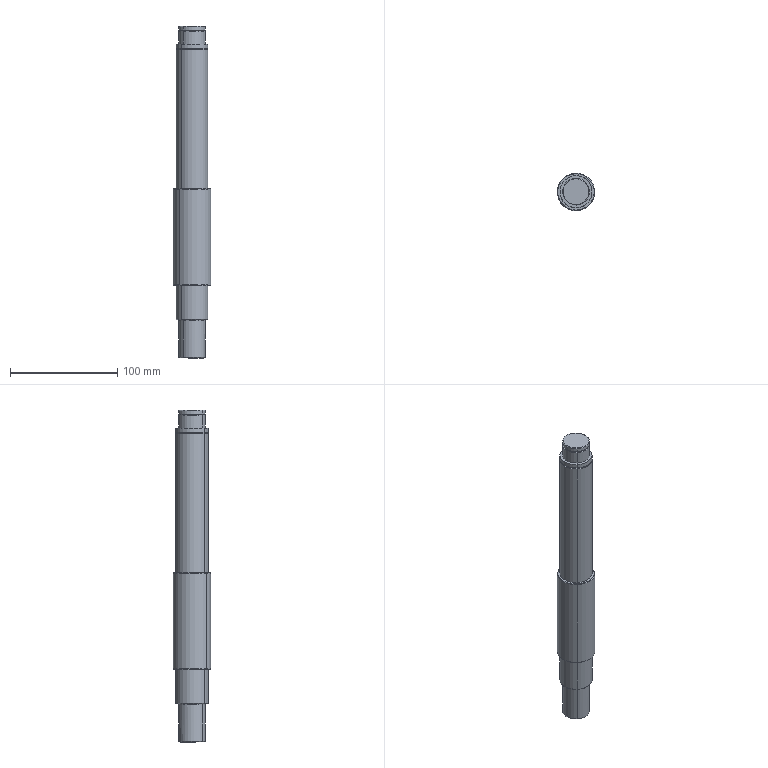Component | SolidWorks | -TractorDriveShaft-1 | 1 solid | 49 faces | box 35 x 35 x 310 mm | volume 226207 mm3 | cylinder 22 | plane 16 | cone 9 | torus 2 | commonest cylinder face diameters 25 x6 30 x6 8 x4 35 x2 27 x2 22.6 x2
build123d program:
from build123d import *

# Parameters (mm, degrees)
CUT_EXTRUDE2_DEPTH = 4.5
CHAMFER1_SIZE      = 0.5
CHAMFER3_SIZE      = 0.5
CUT_EXTRUDE4_DEPTH = 4
CHAMFER4_SIZE      = 0.5
FILLET1_R          = 0.5
CHAMFER5_SIZE      = 0.5
CHAMFER6_SIZE      = 0.5


with BuildPart() as part:
    # Sketch1 → Revolve1 (revolve)
    with BuildSketch(Plane.XY, mode=Mode.PRIVATE) as revolve1_sk:
        Polygon((0, 0), (0, 12.5), (3.8, 12.5), (3.8, 11.3), (5, 11.3), (5, 12.5), (17, 12.5), (17, 15), (20.8, 15), (20.8, 13.5), (22, 13.5), (22, 15), (152, 15), (152, 17.5), (242, 17.5), (242, 15), (274.5, 15), (274.5, 12.5), (310, 12.5), (310, 0), align=None)
    revolve(revolve1_sk.sketch.rotate(Axis((-432.237, 0, 0), (1, 0, 0)), 90), axis=Axis((-432.237, 0, 0), (1, 0, 0)))

    # Sketch3 → Cut-Extrude2 (cut)
    with BuildSketch(Plane.XY.offset(15)):
        with BuildLine():
            Line((28.5, 4), (115.5, 4))
            ThreePointArc((115.5, 4), (119.5, 0), (115.5, -4))
            Line((115.5, -4), (28.5, -4))
            ThreePointArc((28.5, -4), (24.5, 0), (28.5, 4))
        make_face()
    extrude(amount=-CUT_EXTRUDE2_DEPTH, mode=Mode.SUBTRACT)

    # Chamfer1
    chamfer1_edges = [part.edges().sort_by_distance(p)[0] for p in [
        (310, 0, -12.5),
    ]]
    chamfer(chamfer1_edges, length=CHAMFER1_SIZE)

    # Chamfer3
    chamfer3_edges = [part.edges().sort_by_distance(p)[0] for p in [
        (152, 0, -17.5),
    ]]
    chamfer(chamfer3_edges, length=CHAMFER3_SIZE)

    # Sketch5 → Cut-Extrude4 (cut)
    with BuildSketch(Plane.XY.offset(12.5)):
        with BuildLine():
            Line((280, 4), (350, 4))
            ThreePointArc((350, 4), (354, 0), (350, -4))
            Line((350, -4), (280, -4))
            ThreePointArc((280, -4), (276, 0), (280, 4))
        make_face()
    extrude(amount=-CUT_EXTRUDE4_DEPTH, mode=Mode.SUBTRACT)

    # Chamfer4
    chamfer4_edges = [part.edges().sort_by_distance(p)[0] for p in [
        (0, 0, -12.5),
    ]]
    chamfer(chamfer4_edges, length=CHAMFER4_SIZE)

    # Fillet1
    fillet1_edges = [part.edges().sort_by_distance(p)[0] for p in [
        (274.5, 0, -12.5),
    ]]
    fillet(fillet1_edges, radius=FILLET1_R)

    # Chamfer5
    chamfer5_edges = [part.edges().sort_by_distance(p)[0] for p in [
        (242, 0, -17.5),
    ]]
    chamfer(chamfer5_edges, length=CHAMFER5_SIZE)

    # Chamfer6
    chamfer6_edges = [part.edges().sort_by_distance(p)[0] for p in [
        (274.5, 0, -15),
    ]]
    chamfer(chamfer6_edges, length=CHAMFER6_SIZE)


solid = part.part

# Placed as in the assembly
solid = solid.moved(Location((205, 1094.5, 157), (-90, 40.528, 90)))